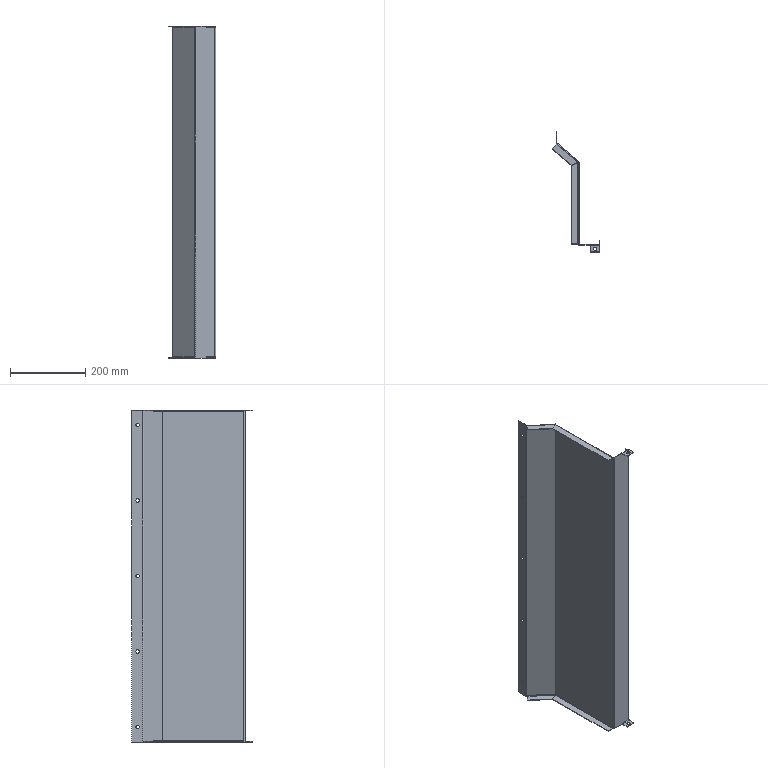Component | SolidWorks | ProtectivePlate-1 | 1 solid | 114 faces | volume 530529 mm3 | plane 76 | cylinder 34 | spline 4 | commonest cylinder face diameters 9 x14 3 x10 6 x10